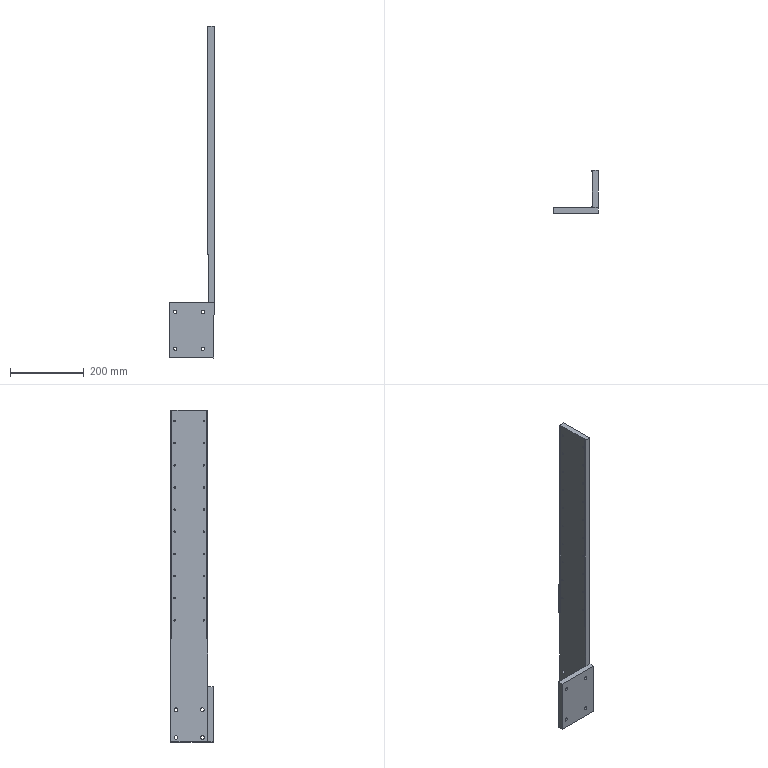Component | SolidWorks | LinearRailConnectionPlate-1 | 1 solid | 124 faces | box 120.97 x 115 x 900.02 mm | volume 1615812 mm3 | cylinder 64 | cone 40 | plane 20 | commonest cylinder face diameters 4 x40 10 x8 15 x8 9 x8
build123d program:
from build123d import *

# Parameters (mm, degrees)
SKETCH1_W                                       = 900
SKETCH1_H                                       = 100
BOSS_EXTRUDE1_DEPTH                             = 15
BOSS_EXTRUDE2_DEPTH                             = 105
BOSS_EXTRUDE2_DEPTH_BACK                        = 15
SKETCH2_W                                       = 150
SKETCH2_H                                       = 15
M8_HEX_SOCKET_HEAD_CAP_SCREW_CBORE1_D           = 9
M8_HEX_SOCKET_HEAD_CAP_SCREW_CBORE1_DEPTH       = 25
M8_HEX_SOCKET_HEAD_CAP_SCREW_CBORE1_CBORE_D     = 15
M8_HEX_SOCKET_HEAD_CAP_SCREW_CBORE1_CBORE_DEPTH = 9
M8_HEX_SOCKET_HEAD_CAP_SCREW_CBORE1_TIP         = 2.704
M10_TAPPED_HOLE1_D                              = 10
M10_TAPPED_HOLE1_DEPTH                          = 24.5
M10_TAPPED_HOLE1_TIP                            = 3.004
LPATTERN1_COUNT                                 = 10
LPATTERN1_PITCH                                 = 60
SKETCH12_W                                      = 3
SKETCH12_H                                      = 2.971
BOSS_EXTRUDE3_DEPTH                             = 620


with BuildPart() as part:
    # Sketch1 → Boss-Extrude1 (new body)
    with BuildSketch(Plane(origin=(0, 0, 0), x_dir=(0, 0, -1), z_dir=(1, 0, 0))):
        Rectangle(SKETCH1_W, SKETCH1_H)
    extrude(amount=BOSS_EXTRUDE1_DEPTH)

    # Sketch2 → Boss-Extrude2 (add, two sides: drawn at the far end of the back side and taken through both)
    with BuildSketch(Plane(origin=(15, 0, 0), x_dir=(0, 0, -1), z_dir=(1, 0, 0)).offset(-BOSS_EXTRUDE2_DEPTH_BACK)):
        with Locations((375, 57.5)):
            Rectangle(SKETCH2_W, SKETCH2_H)
    extrude(amount=BOSS_EXTRUDE2_DEPTH + BOSS_EXTRUDE2_DEPTH_BACK)

    # M8 Hex Socket Head Cap Screw CBORE1
    with Locations(Plane(origin=(0, 50, 0), x_dir=(-1, 0, 0), z_dir=(0, -1, 0))):
        with Locations((-30, 325), (-105, 325), (-105, 425), (-30, 425)):
            CounterBoreHole(M8_HEX_SOCKET_HEAD_CAP_SCREW_CBORE1_D / 2, M8_HEX_SOCKET_HEAD_CAP_SCREW_CBORE1_CBORE_D / 2, M8_HEX_SOCKET_HEAD_CAP_SCREW_CBORE1_CBORE_DEPTH, depth=M8_HEX_SOCKET_HEAD_CAP_SCREW_CBORE1_DEPTH)
            with Locations((0, 0, -(M8_HEX_SOCKET_HEAD_CAP_SCREW_CBORE1_DEPTH + M8_HEX_SOCKET_HEAD_CAP_SCREW_CBORE1_TIP / 2))):  # 118° drill point
                Cone(0, M8_HEX_SOCKET_HEAD_CAP_SCREW_CBORE1_D / 2, M8_HEX_SOCKET_HEAD_CAP_SCREW_CBORE1_TIP, mode=Mode.SUBTRACT)

    # M10 Tapped Hole1
    with Locations(Plane(origin=(15, 0, 0), x_dir=(0, 0, -1), z_dir=(1, 0, 0))):
        with Locations((362.5, -35.5), (437.5, -35.5), (437.5, 35.5), (362.5, 35.5)):
            Hole(M10_TAPPED_HOLE1_D / 2, depth=M10_TAPPED_HOLE1_DEPTH)
            with Locations((0, 0, -(M10_TAPPED_HOLE1_DEPTH + M10_TAPPED_HOLE1_TIP / 2))):  # 118° drill point
                Cone(0, M10_TAPPED_HOLE1_D / 2, M10_TAPPED_HOLE1_TIP, mode=Mode.SUBTRACT)

    # Sketch9 → M4 Tapped Hole1 (revolve, cut)
    with BuildSketch(Plane(origin=(15, -39.529, -120), x_dir=(0, 0, -1), z_dir=(0, 1, 0))):
        Polygon((0, 0), (0, 11.302), (2, 10.1), (2, 0), align=None)
    m4_tapped_hole1 = revolve(axis=Axis((21.35, -39.529, -120), (-1, 0, 0)), mode=Mode.SUBTRACT)

    # LPattern1: M4 Tapped Hole1 ×10
    with Locations(*[(0, 0, i * LPATTERN1_PITCH) for i in range(1, LPATTERN1_COUNT)]):
        add(m4_tapped_hole1, mode=Mode.SUBTRACT)

    # Mirror1: M4 Tapped Hole1 across plane
    add(m4_tapped_hole1.mirror(Plane(origin=(0, 0, 0), x_dir=(0, 0, 1), z_dir=(0, -1, 0))), mode=Mode.SUBTRACT)

    # Mirror1 copy 1 sketch → Mirror1 copy 1 (revolve, cut)
    with BuildSketch(Plane(origin=(15, 39.529, -60), x_dir=(0, 0, -1), z_dir=(0, -1, 0))):
        Polygon((0, 0), (0, -11.302), (2, -10.1), (2, 0), align=None)
    revolve(axis=Axis((21.35, 39.529, -60), (1, 0, 0)), mode=Mode.SUBTRACT)

    # Mirror1 copy 2 sketch → Mirror1 copy 2 (revolve, cut)
    with BuildSketch(Plane(origin=(15, 39.529, 0), x_dir=(0, 0, -1), z_dir=(0, -1, 0))):
        Polygon((0, 0), (0, -11.302), (2, -10.1), (2, 0), align=None)
    revolve(axis=Axis((21.35, 39.529, 0), (1, 0, 0)), mode=Mode.SUBTRACT)

    # Mirror1 copy 3 sketch → Mirror1 copy 3 (revolve, cut)
    with BuildSketch(Plane(origin=(15, 39.529, 60), x_dir=(0, 0, -1), z_dir=(0, -1, 0))):
        Polygon((0, 0), (0, -11.302), (2, -10.1), (2, 0), align=None)
    revolve(axis=Axis((21.35, 39.529, 60), (1, 0, 0)), mode=Mode.SUBTRACT)

    # Mirror1 copy 4 sketch → Mirror1 copy 4 (revolve, cut)
    with BuildSketch(Plane(origin=(15, 39.529, 120), x_dir=(0, 0, -1), z_dir=(0, -1, 0))):
        Polygon((0, 0), (0, -11.302), (2, -10.1), (2, 0), align=None)
    revolve(axis=Axis((21.35, 39.529, 120), (1, 0, 0)), mode=Mode.SUBTRACT)

    # Mirror1 copy 5 sketch → Mirror1 copy 5 (revolve, cut)
    with BuildSketch(Plane(origin=(15, 39.529, 180), x_dir=(0, 0, -1), z_dir=(0, -1, 0))):
        Polygon((0, 0), (0, -11.302), (2, -10.1), (2, 0), align=None)
    revolve(axis=Axis((21.35, 39.529, 180), (1, 0, 0)), mode=Mode.SUBTRACT)

    # Mirror1 copy 6 sketch → Mirror1 copy 6 (revolve, cut)
    with BuildSketch(Plane(origin=(15, 39.529, 240), x_dir=(0, 0, -1), z_dir=(0, -1, 0))):
        Polygon((0, 0), (0, -11.302), (2, -10.1), (2, 0), align=None)
    revolve(axis=Axis((21.35, 39.529, 240), (1, 0, 0)), mode=Mode.SUBTRACT)

    # Mirror1 copy 7 sketch → Mirror1 copy 7 (revolve, cut)
    with BuildSketch(Plane(origin=(15, 39.529, 300), x_dir=(0, 0, -1), z_dir=(0, -1, 0))):
        Polygon((0, 0), (0, -11.302), (2, -10.1), (2, 0), align=None)
    revolve(axis=Axis((21.35, 39.529, 300), (1, 0, 0)), mode=Mode.SUBTRACT)

    # Mirror1 copy 8 sketch → Mirror1 copy 8 (revolve, cut)
    with BuildSketch(Plane(origin=(15, 39.529, 360), x_dir=(0, 0, -1), z_dir=(0, -1, 0))):
        Polygon((0, 0), (0, -11.302), (2, -10.1), (2, 0), align=None)
    revolve(axis=Axis((21.35, 39.529, 360), (1, 0, 0)), mode=Mode.SUBTRACT)

    # Mirror1 copy 9 sketch → Mirror1 copy 9 (revolve, cut)
    with BuildSketch(Plane(origin=(15, 39.529, 420), x_dir=(0, 0, -1), z_dir=(0, -1, 0))):
        Polygon((0, 0), (0, -11.302), (2, -10.1), (2, 0), align=None)
    revolve(axis=Axis((21.35, 39.529, 420), (1, 0, 0)), mode=Mode.SUBTRACT)

    # Sketch12 → Boss-Extrude3 (add)
    with BuildSketch(Plane.XY.offset(450)):
        with Locations((16.5, -48.514)):
            Rectangle(SKETCH12_W, SKETCH12_H)
    boss_extrude3 = extrude(amount=-BOSS_EXTRUDE3_DEPTH)

    # Mirror2: Boss-Extrude3 across plane
    add(boss_extrude3.mirror(Plane(origin=(0, 0, 0), x_dir=(0, 0, 1), z_dir=(0, -1, 0))))


solid = part.part

# Placed as in the assembly
solid = solid.moved(Location((-26.904, 871.583, 941.327), (0, 0.0619, -180)))